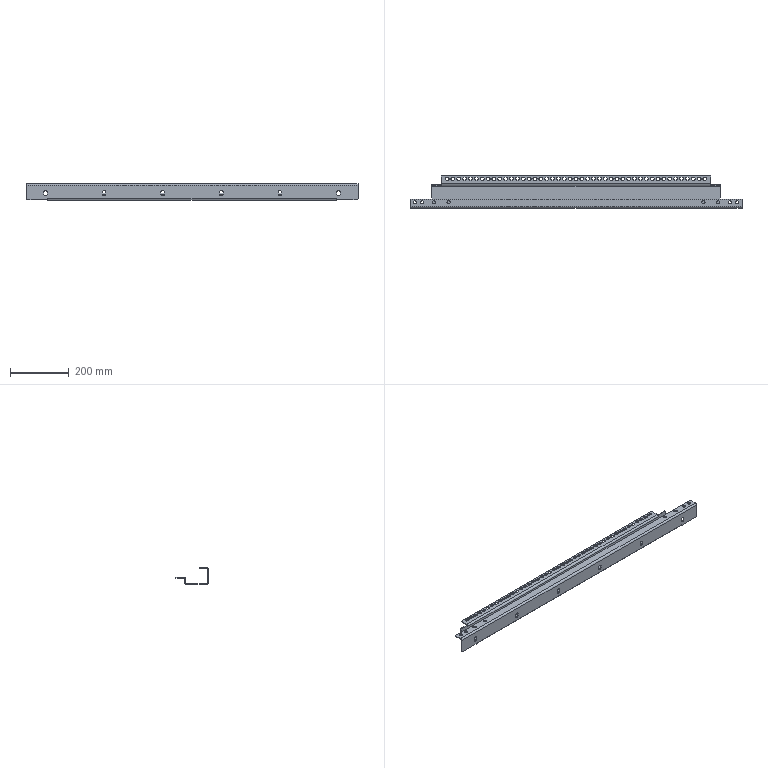Component | SolidWorks | SidePanelAssembly-1_HBSW.001.004SideBottomBeam-1 | 1 solid | 266 faces | volume 619231 mm3 | plane 140 | cylinder 126 | commonest cylinder face diameters 9 x90 11 x16 12 x16 6 x4